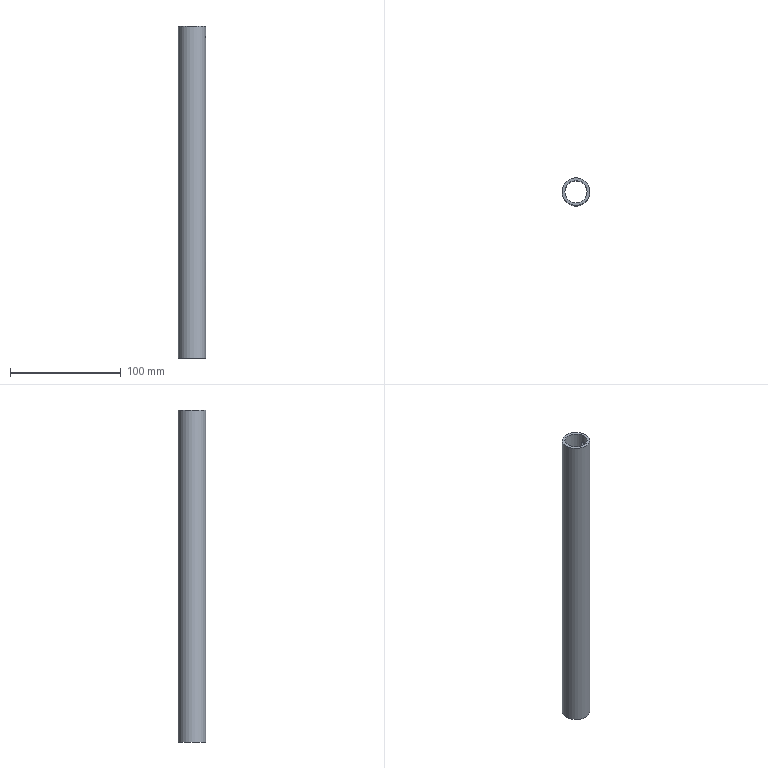Component | NX | SUPPORT_ROD_3 | 1 solid | 5 faces | volume 52955 mm3 | cylinder 3 | plane 2 | commonest cylinder face diameters 25 x1 20 x1 5.5 x1